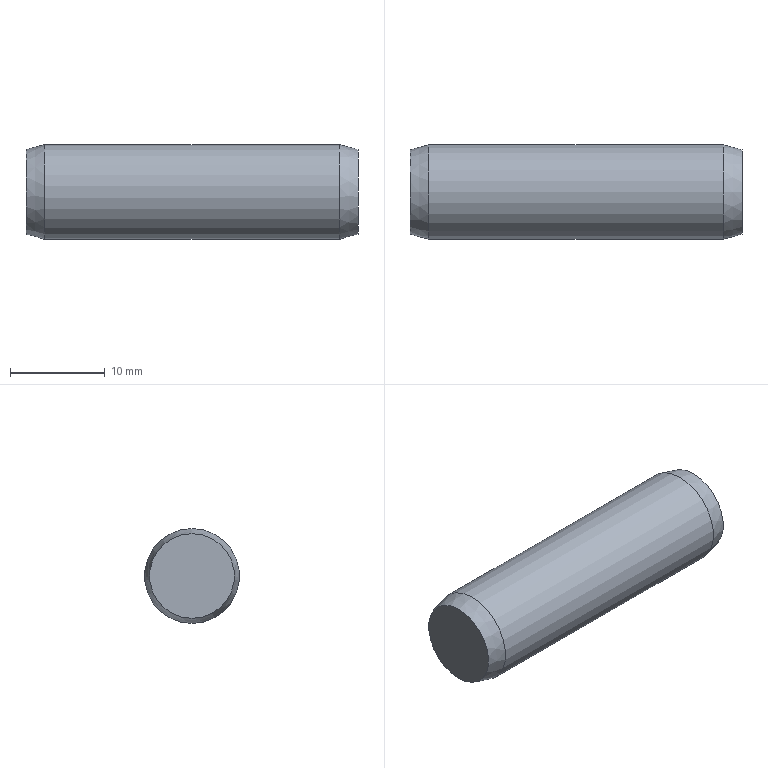Component | NX | GB-T119_1-2000_10X35 | 1 solid | 5 faces | box 35 x 10 x 10 mm | volume 2716 mm3 | plane 2 | cone 2 | cylinder 1 | commonest cylinder face diameters 10 x1
STEP:
#1=CARTESIAN_POINT('',(0.,0.,0.));
#2=DIRECTION('',(0.,0.,1.));
#3=DIRECTION('',(1.,0.,0.));
#4=AXIS2_PLACEMENT_3D('',#1,#2,#3);
#5=CARTESIAN_POINT('',(39.,-65.,193.977));
#6=VERTEX_POINT('',#5);
#7=CARTESIAN_POINT('',(39.,-65.,189.513));
#8=DIRECTION('',(-1.,0.,0.));
#9=DIRECTION('',(0.,0.,1.));
#10=AXIS2_PLACEMENT_3D('',#7,#8,#9);
#11=CIRCLE('',#10,4.464);
#12=CARTESIAN_POINT('',(39.,-65.,189.513));
#13=DIRECTION('',(-1.,0.,0.));
#14=DIRECTION('',(0.,0.,1.));
#15=AXIS2_PLACEMENT_3D('',#12,#13,#14);
#16=PLANE('',#15);
#17=CARTESIAN_POINT('',(0.,0.));
#18=DIRECTION('',(1.,0.));
#19=AXIS2_PLACEMENT_2D('',#17,#18);
#20=CIRCLE('',#19,4.464);
#21=(GEOMETRIC_REPRESENTATION_CONTEXT(2)PARAMETRIC_REPRESENTATION_CONTEXT()REPRESENTATION_CONTEXT('',''));
#22=DEFINITIONAL_REPRESENTATION('',(#20),#21);
#23=PCURVE('',#16,#22);
#24=CARTESIAN_POINT('',(39.,-65.,189.513));
#25=DIRECTION('',(1.,0.,0.));
#26=DIRECTION('',(0.,0.,-1.));
#27=AXIS2_PLACEMENT_3D('',#24,#25,#26);
#28=CONICAL_SURFACE('',#27,4.464,0.2618);
#29=CARTESIAN_POINT('',(9.425,0.));
#30=DIRECTION('',(-1.,0.));
#31=VECTOR('',#30,1.);
#32=LINE('',#29,#31);
#33=(GEOMETRIC_REPRESENTATION_CONTEXT(2)PARAMETRIC_REPRESENTATION_CONTEXT()REPRESENTATION_CONTEXT('',''));
#34=DEFINITIONAL_REPRESENTATION('',(#32),#33);
#35=PCURVE('',#28,#34);
#36=SURFACE_CURVE('',#11,(#23,#35),.PCURVE_S1.);
#37=EDGE_CURVE('',#6,#6,#36,.T.);
#38=ORIENTED_EDGE('',*,*,#37,.T.);
#39=EDGE_LOOP('',(#38));
#40=FACE_BOUND('',#39,.T.);
#41=ADVANCED_FACE('',(#40),#16,.T.);
#42=CARTESIAN_POINT('',(41.,-65.,194.513));
#43=VERTEX_POINT('',#42);
#44=CARTESIAN_POINT('',(41.,-65.,189.513));
#45=DIRECTION('',(-1.,0.,0.));
#46=DIRECTION('',(0.,0.,1.));
#47=AXIS2_PLACEMENT_3D('',#44,#45,#46);
#48=CIRCLE('',#47,5.);
#49=CARTESIAN_POINT('',(9.425,2.));
#50=DIRECTION('',(-1.,0.));
#51=VECTOR('',#50,1.);
#52=LINE('',#49,#51);
#53=(GEOMETRIC_REPRESENTATION_CONTEXT(2)PARAMETRIC_REPRESENTATION_CONTEXT()REPRESENTATION_CONTEXT('',''));
#54=DEFINITIONAL_REPRESENTATION('',(#52),#53);
#55=PCURVE('',#28,#54);
#56=CARTESIAN_POINT('',(74.,-65.,189.513));
#57=DIRECTION('',(-1.,0.,0.));
#58=DIRECTION('',(0.,0.,1.));
#59=AXIS2_PLACEMENT_3D('',#56,#57,#58);
#60=CYLINDRICAL_SURFACE('',#59,5.);
#61=CARTESIAN_POINT('',(0.,33.));
#62=DIRECTION('',(1.,0.));
#63=VECTOR('',#62,1.);
#64=LINE('',#61,#63);
#65=(GEOMETRIC_REPRESENTATION_CONTEXT(2)PARAMETRIC_REPRESENTATION_CONTEXT()REPRESENTATION_CONTEXT('',''));
#66=DEFINITIONAL_REPRESENTATION('',(#64),#65);
#67=PCURVE('',#60,#66);
#68=SURFACE_CURVE('',#48,(#55,#67),.PCURVE_S1.);
#69=EDGE_CURVE('',#43,#43,#68,.T.);
#70=ORIENTED_EDGE('',*,*,#69,.T.);
#71=CARTESIAN_POINT('',(39.,-65.,193.977));
#72=CARTESIAN_POINT('',(41.,-65.,194.513));
#73=B_SPLINE_CURVE_WITH_KNOTS('',1,(#71,#72),.UNSPECIFIED.,.F.,.F.,(2,2),(0.,2.071),.PIECEWISE_BEZIER_KNOTS.);
#74=CARTESIAN_POINT('',(3.142,0.));
#75=DIRECTION('',(0.,1.));
#76=VECTOR('',#75,1.);
#77=LINE('',#74,#76);
#78=(GEOMETRIC_REPRESENTATION_CONTEXT(2)PARAMETRIC_REPRESENTATION_CONTEXT()REPRESENTATION_CONTEXT('',''));
#79=DEFINITIONAL_REPRESENTATION('',(#77),#78);
#80=PCURVE('',#28,#79);
#81=CARTESIAN_POINT('',(9.425,0.));
#82=DIRECTION('',(0.,1.));
#83=VECTOR('',#82,1.);
#84=LINE('',#81,#83);
#85=(GEOMETRIC_REPRESENTATION_CONTEXT(2)PARAMETRIC_REPRESENTATION_CONTEXT()REPRESENTATION_CONTEXT('',''));
#86=DEFINITIONAL_REPRESENTATION('',(#84),#85);
#87=PCURVE('',#28,#86);
#88=SEAM_CURVE('',#73,(#80,#87),.PCURVE_S1.);
#89=EDGE_CURVE('',#6,#43,#88,.T.);
#90=ORIENTED_EDGE('',*,*,#89,.F.);
#91=ORIENTED_EDGE('',*,*,#37,.F.);
#92=ORIENTED_EDGE('',*,*,#89,.T.);
#93=EDGE_LOOP('',(#70,#90,#91,#92));
#94=FACE_BOUND('',#93,.T.);
#95=ADVANCED_FACE('',(#94),#28,.T.);
#96=CARTESIAN_POINT('',(72.,-65.,194.513));
#97=VERTEX_POINT('',#96);
#98=CARTESIAN_POINT('',(72.,-65.,189.513));
#99=DIRECTION('',(-1.,0.,0.));
#100=DIRECTION('',(0.,0.,1.));
#101=AXIS2_PLACEMENT_3D('',#98,#99,#100);
#102=CIRCLE('',#101,5.);
#103=CARTESIAN_POINT('',(0.,2.));
#104=DIRECTION('',(1.,0.));
#105=VECTOR('',#104,1.);
#106=LINE('',#103,#105);
#107=(GEOMETRIC_REPRESENTATION_CONTEXT(2)PARAMETRIC_REPRESENTATION_CONTEXT()REPRESENTATION_CONTEXT('',''));
#108=DEFINITIONAL_REPRESENTATION('',(#106),#107);
#109=PCURVE('',#60,#108);
#110=CARTESIAN_POINT('',(72.,-65.,189.513));
#111=DIRECTION('',(-1.,0.,0.));
#112=DIRECTION('',(0.,0.,1.));
#113=AXIS2_PLACEMENT_3D('',#110,#111,#112);
#114=CONICAL_SURFACE('',#113,5.,0.2618);
#115=CARTESIAN_POINT('',(0.,-0.));
#116=DIRECTION('',(1.,0.));
#117=VECTOR('',#116,1.);
#118=LINE('',#115,#117);
#119=(GEOMETRIC_REPRESENTATION_CONTEXT(2)PARAMETRIC_REPRESENTATION_CONTEXT()REPRESENTATION_CONTEXT('',''));
#120=DEFINITIONAL_REPRESENTATION('',(#118),#119);
#121=PCURVE('',#114,#120);
#122=SURFACE_CURVE('',#102,(#109,#121),.PCURVE_S1.);
#123=EDGE_CURVE('',#97,#97,#122,.T.);
#124=ORIENTED_EDGE('',*,*,#123,.T.);
#125=CARTESIAN_POINT('',(72.,-65.,194.513));
#126=CARTESIAN_POINT('',(41.,-65.,194.513));
#127=B_SPLINE_CURVE_WITH_KNOTS('',1,(#125,#126),.UNSPECIFIED.,.F.,.F.,(2,2),(2.,33.),.PIECEWISE_BEZIER_KNOTS.);
#128=CARTESIAN_POINT('',(6.283,0.));
#129=DIRECTION('',(0.,1.));
#130=VECTOR('',#129,1.);
#131=LINE('',#128,#130);
#132=(GEOMETRIC_REPRESENTATION_CONTEXT(2)PARAMETRIC_REPRESENTATION_CONTEXT()REPRESENTATION_CONTEXT('',''));
#133=DEFINITIONAL_REPRESENTATION('',(#131),#132);
#134=PCURVE('',#60,#133);
#135=CARTESIAN_POINT('',(0.,0.));
#136=DIRECTION('',(0.,1.));
#137=VECTOR('',#136,1.);
#138=LINE('',#135,#137);
#139=(GEOMETRIC_REPRESENTATION_CONTEXT(2)PARAMETRIC_REPRESENTATION_CONTEXT()REPRESENTATION_CONTEXT('',''));
#140=DEFINITIONAL_REPRESENTATION('',(#138),#139);
#141=PCURVE('',#60,#140);
#142=SEAM_CURVE('',#127,(#134,#141),.PCURVE_S1.);
#143=EDGE_CURVE('',#97,#43,#142,.T.);
#144=ORIENTED_EDGE('',*,*,#143,.T.);
#145=ORIENTED_EDGE('',*,*,#69,.F.);
#146=ORIENTED_EDGE('',*,*,#143,.F.);
#147=EDGE_LOOP('',(#124,#144,#145,#146));
#148=FACE_BOUND('',#147,.T.);
#149=ADVANCED_FACE('',(#148),#60,.T.);
#150=CARTESIAN_POINT('',(74.,-65.,193.977));
#151=VERTEX_POINT('',#150);
#152=CARTESIAN_POINT('',(74.,-65.,189.513));
#153=DIRECTION('',(-1.,0.,0.));
#154=DIRECTION('',(0.,0.,1.));
#155=AXIS2_PLACEMENT_3D('',#152,#153,#154);
#156=CIRCLE('',#155,4.464);
#157=CARTESIAN_POINT('',(0.,-2.));
#158=DIRECTION('',(1.,0.));
#159=VECTOR('',#158,1.);
#160=LINE('',#157,#159);
#161=(GEOMETRIC_REPRESENTATION_CONTEXT(2)PARAMETRIC_REPRESENTATION_CONTEXT()REPRESENTATION_CONTEXT('',''));
#162=DEFINITIONAL_REPRESENTATION('',(#160),#161);
#163=PCURVE('',#114,#162);
#164=CARTESIAN_POINT('',(74.,-65.,185.048));
#165=DIRECTION('',(1.,0.,0.));
#166=DIRECTION('',(0.,0.,-1.));
#167=AXIS2_PLACEMENT_3D('',#164,#165,#166);
#168=PLANE('',#167);
#169=CARTESIAN_POINT('',(-8.928,0.));
#170=CARTESIAN_POINT('',(-8.928,7.732));
#171=CARTESIAN_POINT('',(-2.232,3.866));
#172=CARTESIAN_POINT('',(4.464,0.));
#173=CARTESIAN_POINT('',(-2.232,-3.866));
#174=CARTESIAN_POINT('',(-8.928,-7.732));
#175=CARTESIAN_POINT('',(-8.928,0.));
#176=(BOUNDED_CURVE()B_SPLINE_CURVE(2,(#169,#170,#171,#172,#173,#174,#175),.UNSPECIFIED.,.T.,.F.)B_SPLINE_CURVE_WITH_KNOTS((1,2,2,2,2,1),(-2.094,0.,2.094,4.189,6.283,8.378),.UNSPECIFIED.)CURVE()GEOMETRIC_REPRESENTATION_ITEM()RATIONAL_B_SPLINE_CURVE((1.,0.5,1.,0.5,1.,0.5,1.))REPRESENTATION_ITEM(''));
#177=(GEOMETRIC_REPRESENTATION_CONTEXT(2)PARAMETRIC_REPRESENTATION_CONTEXT()REPRESENTATION_CONTEXT('',''));
#178=DEFINITIONAL_REPRESENTATION('',(#176),#177);
#179=PCURVE('',#168,#178);
#180=SURFACE_CURVE('',#156,(#163,#179),.PCURVE_S1.);
#181=EDGE_CURVE('',#151,#151,#180,.T.);
#182=ORIENTED_EDGE('',*,*,#181,.T.);
#183=CARTESIAN_POINT('',(74.,-65.,193.977));
#184=CARTESIAN_POINT('',(72.,-65.,194.513));
#185=B_SPLINE_CURVE_WITH_KNOTS('',1,(#183,#184),.UNSPECIFIED.,.F.,.F.,(2,2),(-2.071,-0.),.PIECEWISE_BEZIER_KNOTS.);
#186=CARTESIAN_POINT('',(6.283,0.));
#187=DIRECTION('',(0.,1.));
#188=VECTOR('',#187,1.);
#189=LINE('',#186,#188);
#190=(GEOMETRIC_REPRESENTATION_CONTEXT(2)PARAMETRIC_REPRESENTATION_CONTEXT()REPRESENTATION_CONTEXT('',''));
#191=DEFINITIONAL_REPRESENTATION('',(#189),#190);
#192=PCURVE('',#114,#191);
#193=CARTESIAN_POINT('',(0.,0.));
#194=DIRECTION('',(0.,1.));
#195=VECTOR('',#194,1.);
#196=LINE('',#193,#195);
#197=(GEOMETRIC_REPRESENTATION_CONTEXT(2)PARAMETRIC_REPRESENTATION_CONTEXT()REPRESENTATION_CONTEXT('',''));
#198=DEFINITIONAL_REPRESENTATION('',(#196),#197);
#199=PCURVE('',#114,#198);
#200=SEAM_CURVE('',#185,(#192,#199),.PCURVE_S1.);
#201=EDGE_CURVE('',#151,#97,#200,.T.);
#202=ORIENTED_EDGE('',*,*,#201,.T.);
#203=ORIENTED_EDGE('',*,*,#123,.F.);
#204=ORIENTED_EDGE('',*,*,#201,.F.);
#205=EDGE_LOOP('',(#182,#202,#203,#204));
#206=FACE_BOUND('',#205,.T.);
#207=ADVANCED_FACE('',(#206),#114,.T.);
#208=ORIENTED_EDGE('',*,*,#181,.F.);
#209=EDGE_LOOP('',(#208));
#210=FACE_BOUND('',#209,.T.);
#211=ADVANCED_FACE('',(#210),#168,.T.);
#212=CLOSED_SHELL('',(#41,#95,#149,#207,#211));
#213=MANIFOLD_SOLID_BREP('',#212);
#214=(LENGTH_UNIT()NAMED_UNIT(*)SI_UNIT(.MILLI.,.METRE.));
#215=UNCERTAINTY_MEASURE_WITH_UNIT(LENGTH_MEASURE(0.00001),#214,'','');
#216=(NAMED_UNIT(*)PLANE_ANGLE_UNIT()SI_UNIT($,.RADIAN.));
#217=(NAMED_UNIT(*)SI_UNIT($,.STERADIAN.)SOLID_ANGLE_UNIT());
#218=(GEOMETRIC_REPRESENTATION_CONTEXT(3)GLOBAL_UNCERTAINTY_ASSIGNED_CONTEXT((#215))GLOBAL_UNIT_ASSIGNED_CONTEXT((#214,#216,#217))REPRESENTATION_CONTEXT('',''));
#219=ADVANCED_BREP_SHAPE_REPRESENTATION('',(#4,#213),#218);